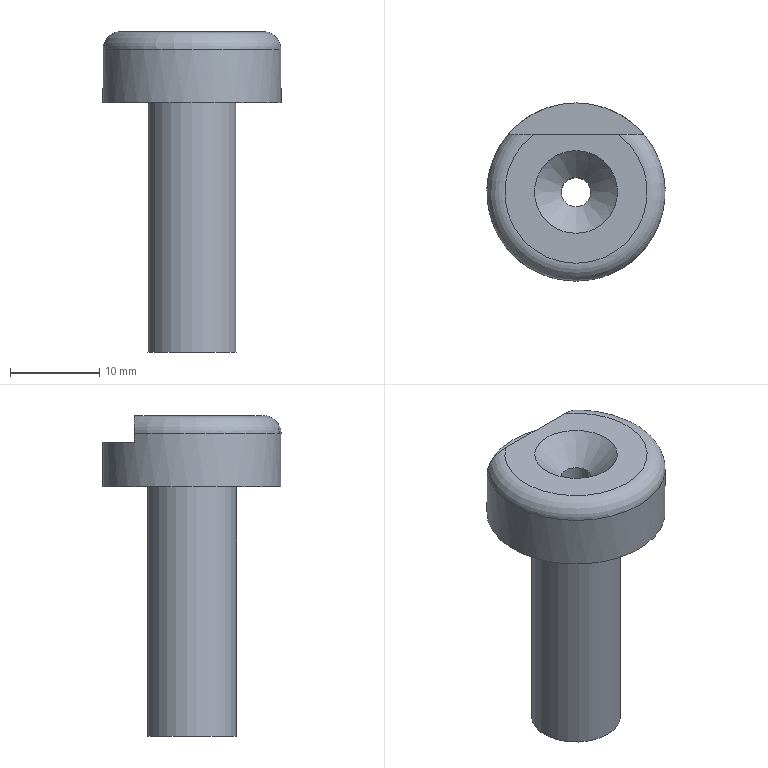Component | NX | DRILL_JIG | 1 solid | 10 faces | box 20 x 20 x 36 mm | volume 4181 mm3 | plane 5 | cylinder 3 | torus 1 | cone 1 | commonest cylinder face diameters 20 x1 10 x1 3.3 x1
STEP:
#1=CARTESIAN_POINT('',(0.,0.,0.));
#2=DIRECTION('',(0.,0.,1.));
#3=DIRECTION('',(1.,0.,0.));
#4=AXIS2_PLACEMENT_3D('',#1,#2,#3);
#5=CARTESIAN_POINT('',(-25.507,208.121,279.845));
#6=VERTEX_POINT('',#5);
#7=CARTESIAN_POINT('',(-25.507,208.121,278.845));
#8=VERTEX_POINT('',#7);
#9=CARTESIAN_POINT('',(-25.507,208.121,281.845));
#10=DIRECTION('',(0.,0.,-1.));
#11=VECTOR('',#10,1.);
#12=LINE('',#9,#11);
#13=CARTESIAN_POINT('',(-17.908,208.121,281.845));
#14=DIRECTION('',(0.,1.,0.));
#15=DIRECTION('',(0.,0.,1.));
#16=AXIS2_PLACEMENT_3D('',#13,#14,#15);
#17=PLANE('',#16);
#18=CARTESIAN_POINT('',(0.,-7.599));
#19=DIRECTION('',(-1.,0.));
#20=VECTOR('',#19,1.);
#21=LINE('',#18,#20);
#22=(GEOMETRIC_REPRESENTATION_CONTEXT(2)PARAMETRIC_REPRESENTATION_CONTEXT()REPRESENTATION_CONTEXT('',''));
#23=DEFINITIONAL_REPRESENTATION('',(#21),#22);
#24=PCURVE('',#17,#23);
#25=CARTESIAN_POINT('',(-17.908,201.621,281.845));
#26=DIRECTION('',(0.,0.,-1.));
#27=DIRECTION('',(0.,1.,0.));
#28=AXIS2_PLACEMENT_3D('',#25,#26,#27);
#29=CYLINDRICAL_SURFACE('',#28,10.);
#30=CARTESIAN_POINT('',(5.42,0.));
#31=DIRECTION('',(0.,1.));
#32=VECTOR('',#31,1.);
#33=LINE('',#30,#32);
#34=(GEOMETRIC_REPRESENTATION_CONTEXT(2)PARAMETRIC_REPRESENTATION_CONTEXT()REPRESENTATION_CONTEXT('',''));
#35=DEFINITIONAL_REPRESENTATION('',(#33),#34);
#36=PCURVE('',#29,#35);
#37=SURFACE_CURVE('',#12,(#24,#36),.PCURVE_S1.);
#38=EDGE_CURVE('',#6,#8,#37,.T.);
#39=ORIENTED_EDGE('',*,*,#38,.F.);
#40=CARTESIAN_POINT('',(-22.572,208.121,281.845));
#41=VERTEX_POINT('',#40);
#42=CARTESIAN_POINT('',(-25.507,208.121,279.845));
#43=CARTESIAN_POINT('',(-25.507,208.121,280.028));
#44=CARTESIAN_POINT('',(-25.473,208.121,280.213));
#45=CARTESIAN_POINT('',(-25.409,208.121,280.385));
#46=CARTESIAN_POINT('',(-25.346,208.121,280.556));
#47=CARTESIAN_POINT('',(-25.252,208.121,280.717));
#48=CARTESIAN_POINT('',(-25.139,208.121,280.86));
#49=CARTESIAN_POINT('',(-24.991,208.121,281.046));
#50=CARTESIAN_POINT('',(-24.807,208.121,281.206));
#51=CARTESIAN_POINT('',(-24.608,208.121,281.334));
#52=CARTESIAN_POINT('',(-24.335,208.121,281.509));
#53=CARTESIAN_POINT('',(-24.027,208.121,281.633));
#54=CARTESIAN_POINT('',(-23.713,208.121,281.713));
#55=CARTESIAN_POINT('',(-23.342,208.121,281.807));
#56=CARTESIAN_POINT('',(-22.955,208.121,281.845));
#57=CARTESIAN_POINT('',(-22.572,208.121,281.845));
#58=B_SPLINE_CURVE_WITH_KNOTS('',3,(#42,#43,#44,#45,#46,#47,#48,#49,#50,#51,#52,#53,#54,#55,#56,#57),.UNSPECIFIED.,.F.,.F.,(4,3,3,3,3,4),(0.,0.1396,0.2785,0.4597,0.7074,1.),.UNSPECIFIED.);
#59=CARTESIAN_POINT('',(-2.,-7.599));
#60=CARTESIAN_POINT('',(-1.817,-7.599));
#61=CARTESIAN_POINT('',(-1.631,-7.565));
#62=CARTESIAN_POINT('',(-1.46,-7.501));
#63=CARTESIAN_POINT('',(-1.289,-7.438));
#64=CARTESIAN_POINT('',(-1.127,-7.344));
#65=CARTESIAN_POINT('',(-0.9843,-7.231));
#66=CARTESIAN_POINT('',(-0.7983,-7.083));
#67=CARTESIAN_POINT('',(-0.6387,-6.899));
#68=CARTESIAN_POINT('',(-0.5103,-6.699));
#69=CARTESIAN_POINT('',(-0.3353,-6.427));
#70=CARTESIAN_POINT('',(-0.2122,-6.119));
#71=CARTESIAN_POINT('',(-0.1322,-5.805));
#72=CARTESIAN_POINT('',(-0.03753,-5.434));
#73=CARTESIAN_POINT('',(0.,-5.047));
#74=CARTESIAN_POINT('',(0.,-4.664));
#75=B_SPLINE_CURVE_WITH_KNOTS('',3,(#59,#60,#61,#62,#63,#64,#65,#66,#67,#68,#69,#70,#71,#72,#73,#74),.UNSPECIFIED.,.F.,.F.,(4,3,3,3,3,4),(0.,0.1396,0.2785,0.4597,0.7074,1.),.UNSPECIFIED.);
#76=(GEOMETRIC_REPRESENTATION_CONTEXT(2)PARAMETRIC_REPRESENTATION_CONTEXT()REPRESENTATION_CONTEXT('',''));
#77=DEFINITIONAL_REPRESENTATION('',(#75),#76);
#78=PCURVE('',#17,#77);
#79=CARTESIAN_POINT('',(-17.908,201.621,279.845));
#80=DIRECTION('',(0.,0.,1.));
#81=DIRECTION('',(0.,-1.,0.));
#82=AXIS2_PLACEMENT_3D('',#79,#80,#81);
#83=TOROIDAL_SURFACE('',#82,8.,2.);
#84=CARTESIAN_POINT('',(4.005,0.));
#85=CARTESIAN_POINT('',(4.005,0.02978));
#86=CARTESIAN_POINT('',(4.004,0.08962));
#87=CARTESIAN_POINT('',(4.002,0.1793));
#88=CARTESIAN_POINT('',(3.999,0.2674));
#89=CARTESIAN_POINT('',(3.994,0.3541));
#90=CARTESIAN_POINT('',(3.988,0.4396));
#91=CARTESIAN_POINT('',(3.981,0.5229));
#92=CARTESIAN_POINT('',(3.973,0.6032));
#93=CARTESIAN_POINT('',(3.964,0.6819));
#94=CARTESIAN_POINT('',(3.954,0.7584));
#95=CARTESIAN_POINT('',(3.943,0.8325));
#96=CARTESIAN_POINT('',(3.932,0.9038));
#97=CARTESIAN_POINT('',(3.92,0.9734));
#98=CARTESIAN_POINT('',(3.907,1.041));
#99=CARTESIAN_POINT('',(3.893,1.107));
#100=CARTESIAN_POINT('',(3.879,1.171));
#101=CARTESIAN_POINT('',(3.864,1.232));
#102=CARTESIAN_POINT('',(3.849,1.292));
#103=CARTESIAN_POINT('',(3.833,1.351));
#104=CARTESIAN_POINT('',(3.816,1.408));
#105=CARTESIAN_POINT('',(3.799,1.464));
#106=CARTESIAN_POINT('',(3.782,1.518));
#107=CARTESIAN_POINT('',(3.77,1.553));
#108=CARTESIAN_POINT('',(3.764,1.571));
#109=B_SPLINE_CURVE_WITH_KNOTS('',3,(#84,#85,#86,#87,#88,#89,#90,#91,#92,#93,#94,#95,#96,#97,#98,#99,#100,#101,#102,#103,#104,#105,#106,#107,#108),.UNSPECIFIED.,.F.,.F.,(4,1,1,1,1,1,1,1,1,1,1,1,1,1,1,1,1,1,1,1,1,1,4),(0.,0.04545,0.09091,0.1364,0.1818,0.2273,0.2727,0.3182,0.3636,0.4091,0.4545,0.5,0.5455,0.5909,0.6364,0.6818,0.7273,0.7727,0.8182,0.8636,0.9091,0.9545,1.),.QUASI_UNIFORM_KNOTS.);
#110=(GEOMETRIC_REPRESENTATION_CONTEXT(2)PARAMETRIC_REPRESENTATION_CONTEXT()REPRESENTATION_CONTEXT('',''));
#111=DEFINITIONAL_REPRESENTATION('',(#109),#110);
#112=PCURVE('',#83,#111);
#113=SURFACE_CURVE('',#58,(#78,#112),.PCURVE_S1.);
#114=EDGE_CURVE('',#6,#41,#113,.T.);
#115=ORIENTED_EDGE('',*,*,#114,.T.);
#116=CARTESIAN_POINT('',(-13.244,208.121,281.845));
#117=VERTEX_POINT('',#116);
#118=CARTESIAN_POINT('',(-17.908,208.121,281.845));
#119=DIRECTION('',(-1.,0.,0.));
#120=VECTOR('',#119,1.);
#121=LINE('',#118,#120);
#122=CARTESIAN_POINT('',(0.,0.));
#123=DIRECTION('',(0.,-1.));
#124=VECTOR('',#123,1.);
#125=LINE('',#122,#124);
#126=(GEOMETRIC_REPRESENTATION_CONTEXT(2)PARAMETRIC_REPRESENTATION_CONTEXT()REPRESENTATION_CONTEXT('',''));
#127=DEFINITIONAL_REPRESENTATION('',(#125),#126);
#128=PCURVE('',#17,#127);
#129=CARTESIAN_POINT('',(-17.908,201.621,281.845));
#130=DIRECTION('',(0.,0.,1.));
#131=DIRECTION('',(0.,-1.,0.));
#132=AXIS2_PLACEMENT_3D('',#129,#130,#131);
#133=PLANE('',#132);
#134=CARTESIAN_POINT('',(-6.5,0.));
#135=DIRECTION('',(0.,-1.));
#136=VECTOR('',#135,1.);
#137=LINE('',#134,#136);
#138=(GEOMETRIC_REPRESENTATION_CONTEXT(2)PARAMETRIC_REPRESENTATION_CONTEXT()REPRESENTATION_CONTEXT('',''));
#139=DEFINITIONAL_REPRESENTATION('',(#137),#138);
#140=PCURVE('',#133,#139);
#141=SURFACE_CURVE('',#121,(#128,#140),.PCURVE_S1.);
#142=EDGE_CURVE('',#117,#41,#141,.T.);
#143=ORIENTED_EDGE('',*,*,#142,.F.);
#144=CARTESIAN_POINT('',(-10.309,208.121,279.845));
#145=VERTEX_POINT('',#144);
#146=CARTESIAN_POINT('',(-13.244,208.121,281.845));
#147=CARTESIAN_POINT('',(-12.586,208.121,281.845));
#148=CARTESIAN_POINT('',(-11.925,208.121,281.739));
#149=CARTESIAN_POINT('',(-10.775,208.121,281.099));
#150=CARTESIAN_POINT('',(-10.309,208.121,280.513));
#151=CARTESIAN_POINT('',(-10.309,208.121,279.845));
#152=B_SPLINE_CURVE_WITH_KNOTS('',3,(#146,#147,#148,#149,#150,#151),.UNSPECIFIED.,.F.,.F.,(4,2,4),(0.,0.5,1.),.UNSPECIFIED.);
#153=CARTESIAN_POINT('',(0.,4.664));
#154=CARTESIAN_POINT('',(0.,5.322));
#155=CARTESIAN_POINT('',(-0.1059,5.983));
#156=CARTESIAN_POINT('',(-0.7454,7.133));
#157=CARTESIAN_POINT('',(-1.331,7.599));
#158=CARTESIAN_POINT('',(-2.,7.599));
#159=B_SPLINE_CURVE_WITH_KNOTS('',3,(#153,#154,#155,#156,#157,#158),.UNSPECIFIED.,.F.,.F.,(4,2,4),(0.,0.5,1.),.UNSPECIFIED.);
#160=(GEOMETRIC_REPRESENTATION_CONTEXT(2)PARAMETRIC_REPRESENTATION_CONTEXT()REPRESENTATION_CONTEXT('',''));
#161=DEFINITIONAL_REPRESENTATION('',(#159),#160);
#162=PCURVE('',#17,#161);
#163=CARTESIAN_POINT('',(8.802,1.571));
#164=CARTESIAN_POINT('',(8.796,1.553));
#165=CARTESIAN_POINT('',(8.784,1.518));
#166=CARTESIAN_POINT('',(8.767,1.464));
#167=CARTESIAN_POINT('',(8.75,1.408));
#168=CARTESIAN_POINT('',(8.733,1.351));
#169=CARTESIAN_POINT('',(8.718,1.292));
#170=CARTESIAN_POINT('',(8.702,1.233));
#171=CARTESIAN_POINT('',(8.688,1.171));
#172=CARTESIAN_POINT('',(8.673,1.108));
#173=CARTESIAN_POINT('',(8.66,1.043));
#174=CARTESIAN_POINT('',(8.647,0.976));
#175=CARTESIAN_POINT('',(8.635,0.9067));
#176=CARTESIAN_POINT('',(8.623,0.8345));
#177=CARTESIAN_POINT('',(8.612,0.7594));
#178=CARTESIAN_POINT('',(8.602,0.6817));
#179=CARTESIAN_POINT('',(8.593,0.6019));
#180=CARTESIAN_POINT('',(8.585,0.5201));
#181=CARTESIAN_POINT('',(8.578,0.4368));
#182=CARTESIAN_POINT('',(8.572,0.3521));
#183=CARTESIAN_POINT('',(8.568,0.2662));
#184=CARTESIAN_POINT('',(8.564,0.179));
#185=CARTESIAN_POINT('',(8.562,0.09049));
#186=CARTESIAN_POINT('',(8.562,0.03038));
#187=CARTESIAN_POINT('',(8.562,0.));
#188=B_SPLINE_CURVE_WITH_KNOTS('',3,(#163,#164,#165,#166,#167,#168,#169,#170,#171,#172,#173,#174,#175,#176,#177,#178,#179,#180,#181,#182,#183,#184,#185,#186,#187),.UNSPECIFIED.,.F.,.F.,(4,1,1,1,1,1,1,1,1,1,1,1,1,1,1,1,1,1,1,1,1,1,4),(0.,0.04545,0.09091,0.1364,0.1818,0.2273,0.2727,0.3182,0.3636,0.4091,0.4545,0.5,0.5455,0.5909,0.6364,0.6818,0.7273,0.7727,0.8182,0.8636,0.9091,0.9545,1.),.QUASI_UNIFORM_KNOTS.);
#189=(GEOMETRIC_REPRESENTATION_CONTEXT(2)PARAMETRIC_REPRESENTATION_CONTEXT()REPRESENTATION_CONTEXT('',''));
#190=DEFINITIONAL_REPRESENTATION('',(#188),#189);
#191=PCURVE('',#83,#190);
#192=SURFACE_CURVE('',#152,(#162,#191),.PCURVE_S1.);
#193=EDGE_CURVE('',#117,#145,#192,.T.);
#194=ORIENTED_EDGE('',*,*,#193,.T.);
#195=CARTESIAN_POINT('',(-10.309,208.121,278.845));
#196=VERTEX_POINT('',#195);
#197=CARTESIAN_POINT('',(-10.309,208.121,281.845));
#198=DIRECTION('',(0.,0.,1.));
#199=VECTOR('',#198,1.);
#200=LINE('',#197,#199);
#201=CARTESIAN_POINT('',(0.,7.599));
#202=DIRECTION('',(1.,0.));
#203=VECTOR('',#202,1.);
#204=LINE('',#201,#203);
#205=(GEOMETRIC_REPRESENTATION_CONTEXT(2)PARAMETRIC_REPRESENTATION_CONTEXT()REPRESENTATION_CONTEXT('',''));
#206=DEFINITIONAL_REPRESENTATION('',(#204),#205);
#207=PCURVE('',#17,#206);
#208=CARTESIAN_POINT('',(0.8632,0.));
#209=DIRECTION('',(0.,-1.));
#210=VECTOR('',#209,1.);
#211=LINE('',#208,#210);
#212=(GEOMETRIC_REPRESENTATION_CONTEXT(2)PARAMETRIC_REPRESENTATION_CONTEXT()REPRESENTATION_CONTEXT('',''));
#213=DEFINITIONAL_REPRESENTATION('',(#211),#212);
#214=PCURVE('',#29,#213);
#215=SURFACE_CURVE('',#200,(#207,#214),.PCURVE_S1.);
#216=EDGE_CURVE('',#196,#145,#215,.T.);
#217=ORIENTED_EDGE('',*,*,#216,.F.);
#218=CARTESIAN_POINT('',(-17.908,208.121,278.845));
#219=DIRECTION('',(1.,0.,0.));
#220=VECTOR('',#219,1.);
#221=LINE('',#218,#220);
#222=CARTESIAN_POINT('',(-3.,0.));
#223=DIRECTION('',(0.,1.));
#224=VECTOR('',#223,1.);
#225=LINE('',#222,#224);
#226=(GEOMETRIC_REPRESENTATION_CONTEXT(2)PARAMETRIC_REPRESENTATION_CONTEXT()REPRESENTATION_CONTEXT('',''));
#227=DEFINITIONAL_REPRESENTATION('',(#225),#226);
#228=PCURVE('',#17,#227);
#229=CARTESIAN_POINT('',(-17.908,201.621,278.845));
#230=DIRECTION('',(0.,0.,1.));
#231=DIRECTION('',(0.,-1.,0.));
#232=AXIS2_PLACEMENT_3D('',#229,#230,#231);
#233=PLANE('',#232);
#234=CARTESIAN_POINT('',(-6.5,0.));
#235=DIRECTION('',(0.,1.));
#236=VECTOR('',#235,1.);
#237=LINE('',#234,#236);
#238=(GEOMETRIC_REPRESENTATION_CONTEXT(2)PARAMETRIC_REPRESENTATION_CONTEXT()REPRESENTATION_CONTEXT('',''));
#239=DEFINITIONAL_REPRESENTATION('',(#237),#238);
#240=PCURVE('',#233,#239);
#241=SURFACE_CURVE('',#221,(#228,#240),.PCURVE_S1.);
#242=EDGE_CURVE('',#8,#196,#241,.T.);
#243=ORIENTED_EDGE('',*,*,#242,.F.);
#244=EDGE_LOOP('',(#39,#115,#143,#194,#217,#243));
#245=FACE_BOUND('',#244,.T.);
#246=ADVANCED_FACE('',(#245),#17,.T.);
#247=CARTESIAN_POINT('',(-17.908,196.971,281.845));
#248=VERTEX_POINT('',#247);
#249=CARTESIAN_POINT('',(-17.908,201.621,281.845));
#250=DIRECTION('',(0.,0.,-1.));
#251=DIRECTION('',(0.,-1.,0.));
#252=AXIS2_PLACEMENT_3D('',#249,#250,#251);
#253=CIRCLE('',#252,4.65);
#254=CARTESIAN_POINT('',(4.65,0.));
#255=CARTESIAN_POINT('',(4.65,-8.054));
#256=CARTESIAN_POINT('',(-2.325,-4.027));
#257=CARTESIAN_POINT('',(-9.3,-0.));
#258=CARTESIAN_POINT('',(-2.325,4.027));
#259=CARTESIAN_POINT('',(4.65,8.054));
#260=CARTESIAN_POINT('',(4.65,0.));
#261=(BOUNDED_CURVE()B_SPLINE_CURVE(2,(#254,#255,#256,#257,#258,#259,#260),.UNSPECIFIED.,.T.,.F.)B_SPLINE_CURVE_WITH_KNOTS((1,2,2,2,2,1),(-2.094,0.,2.094,4.189,6.283,8.378),.UNSPECIFIED.)CURVE()GEOMETRIC_REPRESENTATION_ITEM()RATIONAL_B_SPLINE_CURVE((1.,0.5,1.,0.5,1.,0.5,1.))REPRESENTATION_ITEM(''));
#262=(GEOMETRIC_REPRESENTATION_CONTEXT(2)PARAMETRIC_REPRESENTATION_CONTEXT()REPRESENTATION_CONTEXT('',''));
#263=DEFINITIONAL_REPRESENTATION('',(#261),#262);
#264=PCURVE('',#133,#263);
#265=CARTESIAN_POINT('',(-17.908,201.621,278.845));
#266=DIRECTION('',(0.,0.,1.));
#267=DIRECTION('',(0.,-1.,0.));
#268=AXIS2_PLACEMENT_3D('',#265,#266,#267);
#269=CONICAL_SURFACE('',#268,1.65,0.7854);
#270=CARTESIAN_POINT('',(6.283,3.));
#271=DIRECTION('',(-1.,0.));
#272=VECTOR('',#271,1.);
#273=LINE('',#270,#272);
#274=(GEOMETRIC_REPRESENTATION_CONTEXT(2)PARAMETRIC_REPRESENTATION_CONTEXT()REPRESENTATION_CONTEXT('',''));
#275=DEFINITIONAL_REPRESENTATION('',(#273),#274);
#276=PCURVE('',#269,#275);
#277=SURFACE_CURVE('',#253,(#264,#276),.PCURVE_S1.);
#278=EDGE_CURVE('',#248,#248,#277,.T.);
#279=ORIENTED_EDGE('',*,*,#278,.T.);
#280=EDGE_LOOP('',(#279));
#281=FACE_BOUND('',#280,.T.);
#282=ORIENTED_EDGE('',*,*,#142,.T.);
#283=CARTESIAN_POINT('',(-17.908,201.621,281.845));
#284=DIRECTION('',(0.,0.,1.));
#285=DIRECTION('',(0.,-1.,0.));
#286=AXIS2_PLACEMENT_3D('',#283,#284,#285);
#287=CIRCLE('',#286,8.);
#288=CARTESIAN_POINT('',(0.,0.));
#289=DIRECTION('',(1.,0.));
#290=AXIS2_PLACEMENT_2D('',#288,#289);
#291=CIRCLE('',#290,8.);
#292=(GEOMETRIC_REPRESENTATION_CONTEXT(2)PARAMETRIC_REPRESENTATION_CONTEXT()REPRESENTATION_CONTEXT('',''));
#293=DEFINITIONAL_REPRESENTATION('',(#291),#292);
#294=PCURVE('',#133,#293);
#295=CARTESIAN_POINT('',(0.,1.571));
#296=DIRECTION('',(1.,-0.));
#297=VECTOR('',#296,1.);
#298=LINE('',#295,#297);
#299=(GEOMETRIC_REPRESENTATION_CONTEXT(2)PARAMETRIC_REPRESENTATION_CONTEXT()REPRESENTATION_CONTEXT('',''));
#300=DEFINITIONAL_REPRESENTATION('',(#298),#299);
#301=PCURVE('',#83,#300);
#302=SURFACE_CURVE('',#287,(#294,#301),.PCURVE_S1.);
#303=EDGE_CURVE('',#41,#117,#302,.T.);
#304=ORIENTED_EDGE('',*,*,#303,.T.);
#305=EDGE_LOOP('',(#282,#304));
#306=FACE_BOUND('',#305,.T.);
#307=ADVANCED_FACE('',(#281,#306),#133,.T.);
#308=ORIENTED_EDGE('',*,*,#216,.T.);
#309=CARTESIAN_POINT('',(-17.908,201.621,279.845));
#310=DIRECTION('',(0.,0.,-1.));
#311=DIRECTION('',(0.,-1.,0.));
#312=AXIS2_PLACEMENT_3D('',#309,#310,#311);
#313=CIRCLE('',#312,10.);
#314=CARTESIAN_POINT('',(-3.142,2.));
#315=DIRECTION('',(1.,0.));
#316=VECTOR('',#315,1.);
#317=LINE('',#314,#316);
#318=(GEOMETRIC_REPRESENTATION_CONTEXT(2)PARAMETRIC_REPRESENTATION_CONTEXT()REPRESENTATION_CONTEXT('',''));
#319=DEFINITIONAL_REPRESENTATION('',(#317),#318);
#320=PCURVE('',#29,#319);
#321=CARTESIAN_POINT('',(12.566,0.));
#322=DIRECTION('',(-1.,0.));
#323=VECTOR('',#322,1.);
#324=LINE('',#321,#323);
#325=(GEOMETRIC_REPRESENTATION_CONTEXT(2)PARAMETRIC_REPRESENTATION_CONTEXT()REPRESENTATION_CONTEXT('',''));
#326=DEFINITIONAL_REPRESENTATION('',(#324),#325);
#327=PCURVE('',#83,#326);
#328=SURFACE_CURVE('',#313,(#320,#327),.PCURVE_S1.);
#329=EDGE_CURVE('',#145,#6,#328,.T.);
#330=ORIENTED_EDGE('',*,*,#329,.T.);
#331=ORIENTED_EDGE('',*,*,#38,.T.);
#332=CARTESIAN_POINT('',(-17.908,211.621,278.845));
#333=VERTEX_POINT('',#332);
#334=CARTESIAN_POINT('',(-17.908,201.621,278.845));
#335=DIRECTION('',(0.,0.,-1.));
#336=DIRECTION('',(0.,1.,0.));
#337=AXIS2_PLACEMENT_3D('',#334,#335,#336);
#338=CIRCLE('',#337,10.);
#339=CARTESIAN_POINT('',(0.,3.));
#340=DIRECTION('',(1.,0.));
#341=VECTOR('',#340,1.);
#342=LINE('',#339,#341);
#343=(GEOMETRIC_REPRESENTATION_CONTEXT(2)PARAMETRIC_REPRESENTATION_CONTEXT()REPRESENTATION_CONTEXT('',''));
#344=DEFINITIONAL_REPRESENTATION('',(#342),#343);
#345=PCURVE('',#29,#344);
#346=CARTESIAN_POINT('',(-10.,0.));
#347=CARTESIAN_POINT('',(-10.,17.321));
#348=CARTESIAN_POINT('',(5.,8.66));
#349=CARTESIAN_POINT('',(20.,0.));
#350=CARTESIAN_POINT('',(5.,-8.66));
#351=CARTESIAN_POINT('',(-10.,-17.321));
#352=CARTESIAN_POINT('',(-10.,0.));
#353=(BOUNDED_CURVE()B_SPLINE_CURVE(2,(#346,#347,#348,#349,#350,#351,#352),.UNSPECIFIED.,.T.,.F.)B_SPLINE_CURVE_WITH_KNOTS((1,2,2,2,2,1),(-2.094,0.,2.094,4.189,6.283,8.378),.UNSPECIFIED.)CURVE()GEOMETRIC_REPRESENTATION_ITEM()RATIONAL_B_SPLINE_CURVE((1.,0.5,1.,0.5,1.,0.5,1.))REPRESENTATION_ITEM(''));
#354=(GEOMETRIC_REPRESENTATION_CONTEXT(2)PARAMETRIC_REPRESENTATION_CONTEXT()REPRESENTATION_CONTEXT('',''));
#355=DEFINITIONAL_REPRESENTATION('',(#353),#354);
#356=PCURVE('',#233,#355);
#357=SURFACE_CURVE('',#338,(#345,#356),.PCURVE_S1.);
#358=EDGE_CURVE('',#8,#333,#357,.T.);
#359=ORIENTED_EDGE('',*,*,#358,.T.);
#360=CARTESIAN_POINT('',(-17.908,211.621,273.845));
#361=VERTEX_POINT('',#360);
#362=CARTESIAN_POINT('',(-17.908,211.621,278.845));
#363=CARTESIAN_POINT('',(-17.908,211.621,273.845));
#364=B_SPLINE_CURVE_WITH_KNOTS('',1,(#362,#363),.UNSPECIFIED.,.F.,.F.,(2,2),(3.,8.),.PIECEWISE_BEZIER_KNOTS.);
#365=CARTESIAN_POINT('',(6.283,0.));
#366=DIRECTION('',(0.,1.));
#367=VECTOR('',#366,1.);
#368=LINE('',#365,#367);
#369=(GEOMETRIC_REPRESENTATION_CONTEXT(2)PARAMETRIC_REPRESENTATION_CONTEXT()REPRESENTATION_CONTEXT('',''));
#370=DEFINITIONAL_REPRESENTATION('',(#368),#369);
#371=PCURVE('',#29,#370);
#372=CARTESIAN_POINT('',(0.,0.));
#373=DIRECTION('',(0.,1.));
#374=VECTOR('',#373,1.);
#375=LINE('',#372,#374);
#376=(GEOMETRIC_REPRESENTATION_CONTEXT(2)PARAMETRIC_REPRESENTATION_CONTEXT()REPRESENTATION_CONTEXT('',''));
#377=DEFINITIONAL_REPRESENTATION('',(#375),#376);
#378=PCURVE('',#29,#377);
#379=SEAM_CURVE('',#364,(#371,#378),.PCURVE_S1.);
#380=EDGE_CURVE('',#333,#361,#379,.T.);
#381=ORIENTED_EDGE('',*,*,#380,.T.);
#382=CARTESIAN_POINT('',(-17.908,201.621,273.845));
#383=DIRECTION('',(0.,0.,1.));
#384=DIRECTION('',(0.,1.,0.));
#385=AXIS2_PLACEMENT_3D('',#382,#383,#384);
#386=CIRCLE('',#385,10.);
#387=CARTESIAN_POINT('',(6.283,8.));
#388=DIRECTION('',(-1.,0.));
#389=VECTOR('',#388,1.);
#390=LINE('',#387,#389);
#391=(GEOMETRIC_REPRESENTATION_CONTEXT(2)PARAMETRIC_REPRESENTATION_CONTEXT()REPRESENTATION_CONTEXT('',''));
#392=DEFINITIONAL_REPRESENTATION('',(#390),#391);
#393=PCURVE('',#29,#392);
#394=CARTESIAN_POINT('',(-17.908,201.621,273.845));
#395=DIRECTION('',(0.,0.,-1.));
#396=DIRECTION('',(0.,1.,0.));
#397=AXIS2_PLACEMENT_3D('',#394,#395,#396);
#398=PLANE('',#397);
#399=CARTESIAN_POINT('',(10.,0.));
#400=CARTESIAN_POINT('',(10.,-17.321));
#401=CARTESIAN_POINT('',(-5.,-8.66));
#402=CARTESIAN_POINT('',(-20.,-0.));
#403=CARTESIAN_POINT('',(-5.,8.66));
#404=CARTESIAN_POINT('',(10.,17.321));
#405=CARTESIAN_POINT('',(10.,0.));
#406=(BOUNDED_CURVE()B_SPLINE_CURVE(2,(#399,#400,#401,#402,#403,#404,#405),.UNSPECIFIED.,.T.,.F.)B_SPLINE_CURVE_WITH_KNOTS((1,2,2,2,2,1),(-2.094,0.,2.094,4.189,6.283,8.378),.UNSPECIFIED.)CURVE()GEOMETRIC_REPRESENTATION_ITEM()RATIONAL_B_SPLINE_CURVE((1.,0.5,1.,0.5,1.,0.5,1.))REPRESENTATION_ITEM(''));
#407=(GEOMETRIC_REPRESENTATION_CONTEXT(2)PARAMETRIC_REPRESENTATION_CONTEXT()REPRESENTATION_CONTEXT('',''));
#408=DEFINITIONAL_REPRESENTATION('',(#406),#407);
#409=PCURVE('',#398,#408);
#410=SURFACE_CURVE('',#386,(#393,#409),.PCURVE_S1.);
#411=EDGE_CURVE('',#361,#361,#410,.T.);
#412=ORIENTED_EDGE('',*,*,#411,.T.);
#413=ORIENTED_EDGE('',*,*,#380,.F.);
#414=CARTESIAN_POINT('',(-17.908,201.621,278.845));
#415=DIRECTION('',(0.,0.,-1.));
#416=DIRECTION('',(0.,1.,0.));
#417=AXIS2_PLACEMENT_3D('',#414,#415,#416);
#418=CIRCLE('',#417,10.);
#419=CARTESIAN_POINT('',(-6.283,3.));
#420=DIRECTION('',(1.,0.));
#421=VECTOR('',#420,1.);
#422=LINE('',#419,#421);
#423=(GEOMETRIC_REPRESENTATION_CONTEXT(2)PARAMETRIC_REPRESENTATION_CONTEXT()REPRESENTATION_CONTEXT('',''));
#424=DEFINITIONAL_REPRESENTATION('',(#422),#423);
#425=PCURVE('',#29,#424);
#426=CARTESIAN_POINT('',(-10.,0.));
#427=CARTESIAN_POINT('',(-10.,17.321));
#428=CARTESIAN_POINT('',(5.,8.66));
#429=CARTESIAN_POINT('',(20.,0.));
#430=CARTESIAN_POINT('',(5.,-8.66));
#431=CARTESIAN_POINT('',(-10.,-17.321));
#432=CARTESIAN_POINT('',(-10.,0.));
#433=(BOUNDED_CURVE()B_SPLINE_CURVE(2,(#426,#427,#428,#429,#430,#431,#432),.UNSPECIFIED.,.T.,.F.)B_SPLINE_CURVE_WITH_KNOTS((1,2,2,2,2,1),(-2.094,0.,2.094,4.189,6.283,8.378),.UNSPECIFIED.)CURVE()GEOMETRIC_REPRESENTATION_ITEM()RATIONAL_B_SPLINE_CURVE((1.,0.5,1.,0.5,1.,0.5,1.))REPRESENTATION_ITEM(''));
#434=(GEOMETRIC_REPRESENTATION_CONTEXT(2)PARAMETRIC_REPRESENTATION_CONTEXT()REPRESENTATION_CONTEXT('',''));
#435=DEFINITIONAL_REPRESENTATION('',(#433),#434);
#436=PCURVE('',#233,#435);
#437=SURFACE_CURVE('',#418,(#425,#436),.PCURVE_S1.);
#438=EDGE_CURVE('',#333,#196,#437,.T.);
#439=ORIENTED_EDGE('',*,*,#438,.T.);
#440=EDGE_LOOP('',(#308,#330,#331,#359,#381,#412,#413,#439));
#441=FACE_BOUND('',#440,.T.);
#442=ADVANCED_FACE('',(#441),#29,.T.);
#443=CARTESIAN_POINT('',(-17.908,206.621,273.845));
#444=VERTEX_POINT('',#443);
#445=CARTESIAN_POINT('',(-17.908,201.621,273.845));
#446=DIRECTION('',(0.,0.,-1.));
#447=DIRECTION('',(0.,1.,0.));
#448=AXIS2_PLACEMENT_3D('',#445,#446,#447);
#449=CIRCLE('',#448,5.);
#450=CARTESIAN_POINT('',(0.,0.));
#451=DIRECTION('',(1.,0.));
#452=AXIS2_PLACEMENT_2D('',#450,#451);
#453=CIRCLE('',#452,5.);
#454=(GEOMETRIC_REPRESENTATION_CONTEXT(2)PARAMETRIC_REPRESENTATION_CONTEXT()REPRESENTATION_CONTEXT('',''));
#455=DEFINITIONAL_REPRESENTATION('',(#453),#454);
#456=PCURVE('',#398,#455);
#457=CARTESIAN_POINT('',(-17.908,201.621,273.845));
#458=DIRECTION('',(0.,0.,-1.));
#459=DIRECTION('',(0.,1.,0.));
#460=AXIS2_PLACEMENT_3D('',#457,#458,#459);
#461=CYLINDRICAL_SURFACE('',#460,5.);
#462=CARTESIAN_POINT('',(0.,0.));
#463=DIRECTION('',(1.,0.));
#464=VECTOR('',#463,1.);
#465=LINE('',#462,#464);
#466=(GEOMETRIC_REPRESENTATION_CONTEXT(2)PARAMETRIC_REPRESENTATION_CONTEXT()REPRESENTATION_CONTEXT('',''));
#467=DEFINITIONAL_REPRESENTATION('',(#465),#466);
#468=PCURVE('',#461,#467);
#469=SURFACE_CURVE('',#449,(#456,#468),.PCURVE_S1.);
#470=EDGE_CURVE('',#444,#444,#469,.T.);
#471=ORIENTED_EDGE('',*,*,#470,.F.);
#472=EDGE_LOOP('',(#471));
#473=FACE_BOUND('',#472,.T.);
#474=ORIENTED_EDGE('',*,*,#411,.F.);
#475=EDGE_LOOP('',(#474));
#476=FACE_BOUND('',#475,.T.);
#477=ADVANCED_FACE('',(#473,#476),#398,.T.);
#478=ORIENTED_EDGE('',*,*,#358,.F.);
#479=ORIENTED_EDGE('',*,*,#242,.T.);
#480=ORIENTED_EDGE('',*,*,#438,.F.);
#481=EDGE_LOOP('',(#478,#479,#480));
#482=FACE_BOUND('',#481,.T.);
#483=ADVANCED_FACE('',(#482),#233,.T.);
#484=ORIENTED_EDGE('',*,*,#193,.F.);
#485=ORIENTED_EDGE('',*,*,#303,.F.);
#486=ORIENTED_EDGE('',*,*,#114,.F.);
#487=ORIENTED_EDGE('',*,*,#329,.F.);
#488=EDGE_LOOP('',(#484,#485,#486,#487));
#489=FACE_BOUND('',#488,.T.);
#490=ADVANCED_FACE('',(#489),#83,.T.);
#491=CARTESIAN_POINT('',(-17.908,199.971,245.845));
#492=VERTEX_POINT('',#491);
#493=CARTESIAN_POINT('',(-17.908,201.621,245.845));
#494=DIRECTION('',(0.,0.,1.));
#495=DIRECTION('',(0.,-1.,0.));
#496=AXIS2_PLACEMENT_3D('',#493,#494,#495);
#497=CIRCLE('',#496,1.65);
#498=CARTESIAN_POINT('',(-17.908,201.621,245.845));
#499=DIRECTION('',(0.,0.,-1.));
#500=DIRECTION('',(0.,1.,0.));
#501=AXIS2_PLACEMENT_3D('',#498,#499,#500);
#502=PLANE('',#501);
#503=CARTESIAN_POINT('',(-1.65,0.));
#504=CARTESIAN_POINT('',(-1.65,2.858));
#505=CARTESIAN_POINT('',(0.825,1.429));
#506=CARTESIAN_POINT('',(3.3,0.));
#507=CARTESIAN_POINT('',(0.825,-1.429));
#508=CARTESIAN_POINT('',(-1.65,-2.858));
#509=CARTESIAN_POINT('',(-1.65,0.));
#510=(BOUNDED_CURVE()B_SPLINE_CURVE(2,(#503,#504,#505,#506,#507,#508,#509),.UNSPECIFIED.,.T.,.F.)B_SPLINE_CURVE_WITH_KNOTS((1,2,2,2,2,1),(-2.094,0.,2.094,4.189,6.283,8.378),.UNSPECIFIED.)CURVE()GEOMETRIC_REPRESENTATION_ITEM()RATIONAL_B_SPLINE_CURVE((1.,0.5,1.,0.5,1.,0.5,1.))REPRESENTATION_ITEM(''));
#511=(GEOMETRIC_REPRESENTATION_CONTEXT(2)PARAMETRIC_REPRESENTATION_CONTEXT()REPRESENTATION_CONTEXT('',''));
#512=DEFINITIONAL_REPRESENTATION('',(#510),#511);
#513=PCURVE('',#502,#512);
#514=CARTESIAN_POINT('',(-17.908,201.621,245.845));
#515=DIRECTION('',(0.,0.,1.));
#516=DIRECTION('',(0.,-1.,0.));
#517=AXIS2_PLACEMENT_3D('',#514,#515,#516);
#518=CYLINDRICAL_SURFACE('',#517,1.65);
#519=CARTESIAN_POINT('',(0.,0.));
#520=DIRECTION('',(1.,0.));
#521=VECTOR('',#520,1.);
#522=LINE('',#519,#521);
#523=(GEOMETRIC_REPRESENTATION_CONTEXT(2)PARAMETRIC_REPRESENTATION_CONTEXT()REPRESENTATION_CONTEXT('',''));
#524=DEFINITIONAL_REPRESENTATION('',(#522),#523);
#525=PCURVE('',#518,#524);
#526=SURFACE_CURVE('',#497,(#513,#525),.PCURVE_S1.);
#527=EDGE_CURVE('',#492,#492,#526,.T.);
#528=ORIENTED_EDGE('',*,*,#527,.T.);
#529=EDGE_LOOP('',(#528));
#530=FACE_BOUND('',#529,.T.);
#531=CARTESIAN_POINT('',(-17.908,206.621,245.845));
#532=VERTEX_POINT('',#531);
#533=CARTESIAN_POINT('',(-17.908,201.621,245.845));
#534=DIRECTION('',(0.,0.,1.));
#535=DIRECTION('',(0.,1.,0.));
#536=AXIS2_PLACEMENT_3D('',#533,#534,#535);
#537=CIRCLE('',#536,5.);
#538=CARTESIAN_POINT('',(5.,0.));
#539=CARTESIAN_POINT('',(5.,-8.66));
#540=CARTESIAN_POINT('',(-2.5,-4.33));
#541=CARTESIAN_POINT('',(-10.,-0.));
#542=CARTESIAN_POINT('',(-2.5,4.33));
#543=CARTESIAN_POINT('',(5.,8.66));
#544=CARTESIAN_POINT('',(5.,0.));
#545=(BOUNDED_CURVE()B_SPLINE_CURVE(2,(#538,#539,#540,#541,#542,#543,#544),.UNSPECIFIED.,.T.,.F.)B_SPLINE_CURVE_WITH_KNOTS((1,2,2,2,2,1),(-2.094,0.,2.094,4.189,6.283,8.378),.UNSPECIFIED.)CURVE()GEOMETRIC_REPRESENTATION_ITEM()RATIONAL_B_SPLINE_CURVE((1.,0.5,1.,0.5,1.,0.5,1.))REPRESENTATION_ITEM(''));
#546=(GEOMETRIC_REPRESENTATION_CONTEXT(2)PARAMETRIC_REPRESENTATION_CONTEXT()REPRESENTATION_CONTEXT('',''));
#547=DEFINITIONAL_REPRESENTATION('',(#545),#546);
#548=PCURVE('',#502,#547);
#549=CARTESIAN_POINT('',(6.283,28.));
#550=DIRECTION('',(-1.,0.));
#551=VECTOR('',#550,1.);
#552=LINE('',#549,#551);
#553=(GEOMETRIC_REPRESENTATION_CONTEXT(2)PARAMETRIC_REPRESENTATION_CONTEXT()REPRESENTATION_CONTEXT('',''));
#554=DEFINITIONAL_REPRESENTATION('',(#552),#553);
#555=PCURVE('',#461,#554);
#556=SURFACE_CURVE('',#537,(#548,#555),.PCURVE_S1.);
#557=EDGE_CURVE('',#532,#532,#556,.T.);
#558=ORIENTED_EDGE('',*,*,#557,.F.);
#559=EDGE_LOOP('',(#558));
#560=FACE_BOUND('',#559,.T.);
#561=ADVANCED_FACE('',(#530,#560),#502,.T.);
#562=ORIENTED_EDGE('',*,*,#557,.T.);
#563=CARTESIAN_POINT('',(-17.908,206.621,273.845));
#564=CARTESIAN_POINT('',(-17.908,206.621,245.845));
#565=B_SPLINE_CURVE_WITH_KNOTS('',1,(#563,#564),.UNSPECIFIED.,.F.,.F.,(2,2),(0.,28.),.PIECEWISE_BEZIER_KNOTS.);
#566=CARTESIAN_POINT('',(0.,0.));
#567=DIRECTION('',(0.,1.));
#568=VECTOR('',#567,1.);
#569=LINE('',#566,#568);
#570=(GEOMETRIC_REPRESENTATION_CONTEXT(2)PARAMETRIC_REPRESENTATION_CONTEXT()REPRESENTATION_CONTEXT('',''));
#571=DEFINITIONAL_REPRESENTATION('',(#569),#570);
#572=PCURVE('',#461,#571);
#573=CARTESIAN_POINT('',(6.283,0.));
#574=DIRECTION('',(0.,1.));
#575=VECTOR('',#574,1.);
#576=LINE('',#573,#575);
#577=(GEOMETRIC_REPRESENTATION_CONTEXT(2)PARAMETRIC_REPRESENTATION_CONTEXT()REPRESENTATION_CONTEXT('',''));
#578=DEFINITIONAL_REPRESENTATION('',(#576),#577);
#579=PCURVE('',#461,#578);
#580=SEAM_CURVE('',#565,(#572,#579),.PCURVE_S1.);
#581=EDGE_CURVE('',#444,#532,#580,.T.);
#582=ORIENTED_EDGE('',*,*,#581,.F.);
#583=ORIENTED_EDGE('',*,*,#470,.T.);
#584=ORIENTED_EDGE('',*,*,#581,.T.);
#585=EDGE_LOOP('',(#562,#582,#583,#584));
#586=FACE_BOUND('',#585,.T.);
#587=ADVANCED_FACE('',(#586),#461,.T.);
#588=CARTESIAN_POINT('',(-17.908,199.971,278.845));
#589=VERTEX_POINT('',#588);
#590=CARTESIAN_POINT('',(-17.908,201.621,278.845));
#591=DIRECTION('',(0.,0.,1.));
#592=DIRECTION('',(0.,-1.,0.));
#593=AXIS2_PLACEMENT_3D('',#590,#591,#592);
#594=CIRCLE('',#593,1.65);
#595=CARTESIAN_POINT('',(0.,33.));
#596=DIRECTION('',(1.,0.));
#597=VECTOR('',#596,1.);
#598=LINE('',#595,#597);
#599=(GEOMETRIC_REPRESENTATION_CONTEXT(2)PARAMETRIC_REPRESENTATION_CONTEXT()REPRESENTATION_CONTEXT('',''));
#600=DEFINITIONAL_REPRESENTATION('',(#598),#599);
#601=PCURVE('',#518,#600);
#602=CARTESIAN_POINT('',(0.,0.));
#603=DIRECTION('',(1.,0.));
#604=VECTOR('',#603,1.);
#605=LINE('',#602,#604);
#606=(GEOMETRIC_REPRESENTATION_CONTEXT(2)PARAMETRIC_REPRESENTATION_CONTEXT()REPRESENTATION_CONTEXT('',''));
#607=DEFINITIONAL_REPRESENTATION('',(#605),#606);
#608=PCURVE('',#269,#607);
#609=SURFACE_CURVE('',#594,(#601,#608),.PCURVE_S1.);
#610=EDGE_CURVE('',#589,#589,#609,.T.);
#611=ORIENTED_EDGE('',*,*,#610,.F.);
#612=CARTESIAN_POINT('',(-17.908,199.971,245.845));
#613=CARTESIAN_POINT('',(-17.908,199.971,278.845));
#614=B_SPLINE_CURVE_WITH_KNOTS('',1,(#612,#613),.UNSPECIFIED.,.F.,.F.,(2,2),(0.,33.),.PIECEWISE_BEZIER_KNOTS.);
#615=CARTESIAN_POINT('',(0.,0.));
#616=DIRECTION('',(0.,1.));
#617=VECTOR('',#616,1.);
#618=LINE('',#615,#617);
#619=(GEOMETRIC_REPRESENTATION_CONTEXT(2)PARAMETRIC_REPRESENTATION_CONTEXT()REPRESENTATION_CONTEXT('',''));
#620=DEFINITIONAL_REPRESENTATION('',(#618),#619);
#621=PCURVE('',#518,#620);
#622=CARTESIAN_POINT('',(6.283,0.));
#623=DIRECTION('',(0.,1.));
#624=VECTOR('',#623,1.);
#625=LINE('',#622,#624);
#626=(GEOMETRIC_REPRESENTATION_CONTEXT(2)PARAMETRIC_REPRESENTATION_CONTEXT()REPRESENTATION_CONTEXT('',''));
#627=DEFINITIONAL_REPRESENTATION('',(#625),#626);
#628=PCURVE('',#518,#627);
#629=SEAM_CURVE('',#614,(#621,#628),.PCURVE_S1.);
#630=EDGE_CURVE('',#492,#589,#629,.T.);
#631=ORIENTED_EDGE('',*,*,#630,.F.);
#632=ORIENTED_EDGE('',*,*,#527,.T.);
#633=ORIENTED_EDGE('',*,*,#630,.T.);
#634=EDGE_LOOP('',(#611,#631,#632,#633));
#635=FACE_BOUND('',#634,.F.);
#636=ADVANCED_FACE('',(#635),#518,.F.);
#637=ORIENTED_EDGE('',*,*,#278,.T.);
#638=CARTESIAN_POINT('',(-17.908,199.971,278.845));
#639=CARTESIAN_POINT('',(-17.908,196.971,281.845));
#640=B_SPLINE_CURVE_WITH_KNOTS('',1,(#638,#639),.UNSPECIFIED.,.F.,.F.,(2,2),(0.,4.243),.PIECEWISE_BEZIER_KNOTS.);
#641=CARTESIAN_POINT('',(0.,0.));
#642=DIRECTION('',(0.,1.));
#643=VECTOR('',#642,1.);
#644=LINE('',#641,#643);
#645=(GEOMETRIC_REPRESENTATION_CONTEXT(2)PARAMETRIC_REPRESENTATION_CONTEXT()REPRESENTATION_CONTEXT('',''));
#646=DEFINITIONAL_REPRESENTATION('',(#644),#645);
#647=PCURVE('',#269,#646);
#648=CARTESIAN_POINT('',(6.283,0.));
#649=DIRECTION('',(0.,1.));
#650=VECTOR('',#649,1.);
#651=LINE('',#648,#650);
#652=(GEOMETRIC_REPRESENTATION_CONTEXT(2)PARAMETRIC_REPRESENTATION_CONTEXT()REPRESENTATION_CONTEXT('',''));
#653=DEFINITIONAL_REPRESENTATION('',(#651),#652);
#654=PCURVE('',#269,#653);
#655=SEAM_CURVE('',#640,(#647,#654),.PCURVE_S1.);
#656=EDGE_CURVE('',#589,#248,#655,.T.);
#657=ORIENTED_EDGE('',*,*,#656,.F.);
#658=ORIENTED_EDGE('',*,*,#610,.T.);
#659=ORIENTED_EDGE('',*,*,#656,.T.);
#660=EDGE_LOOP('',(#637,#657,#658,#659));
#661=FACE_BOUND('',#660,.F.);
#662=ADVANCED_FACE('',(#661),#269,.F.);
#663=CLOSED_SHELL('',(#246,#307,#442,#477,#483,#490,#561,#587,#636,#662));
#664=MANIFOLD_SOLID_BREP('',#663);
#665=(LENGTH_UNIT()NAMED_UNIT(*)SI_UNIT(.MILLI.,.METRE.));
#666=UNCERTAINTY_MEASURE_WITH_UNIT(LENGTH_MEASURE(0.001),#665,'','');
#667=(NAMED_UNIT(*)PLANE_ANGLE_UNIT()SI_UNIT($,.RADIAN.));
#668=(NAMED_UNIT(*)SI_UNIT($,.STERADIAN.)SOLID_ANGLE_UNIT());
#669=(GEOMETRIC_REPRESENTATION_CONTEXT(3)GLOBAL_UNCERTAINTY_ASSIGNED_CONTEXT((#666))GLOBAL_UNIT_ASSIGNED_CONTEXT((#665,#667,#668))REPRESENTATION_CONTEXT('',''));
#670=ADVANCED_BREP_SHAPE_REPRESENTATION('',(#4,#664),#669);